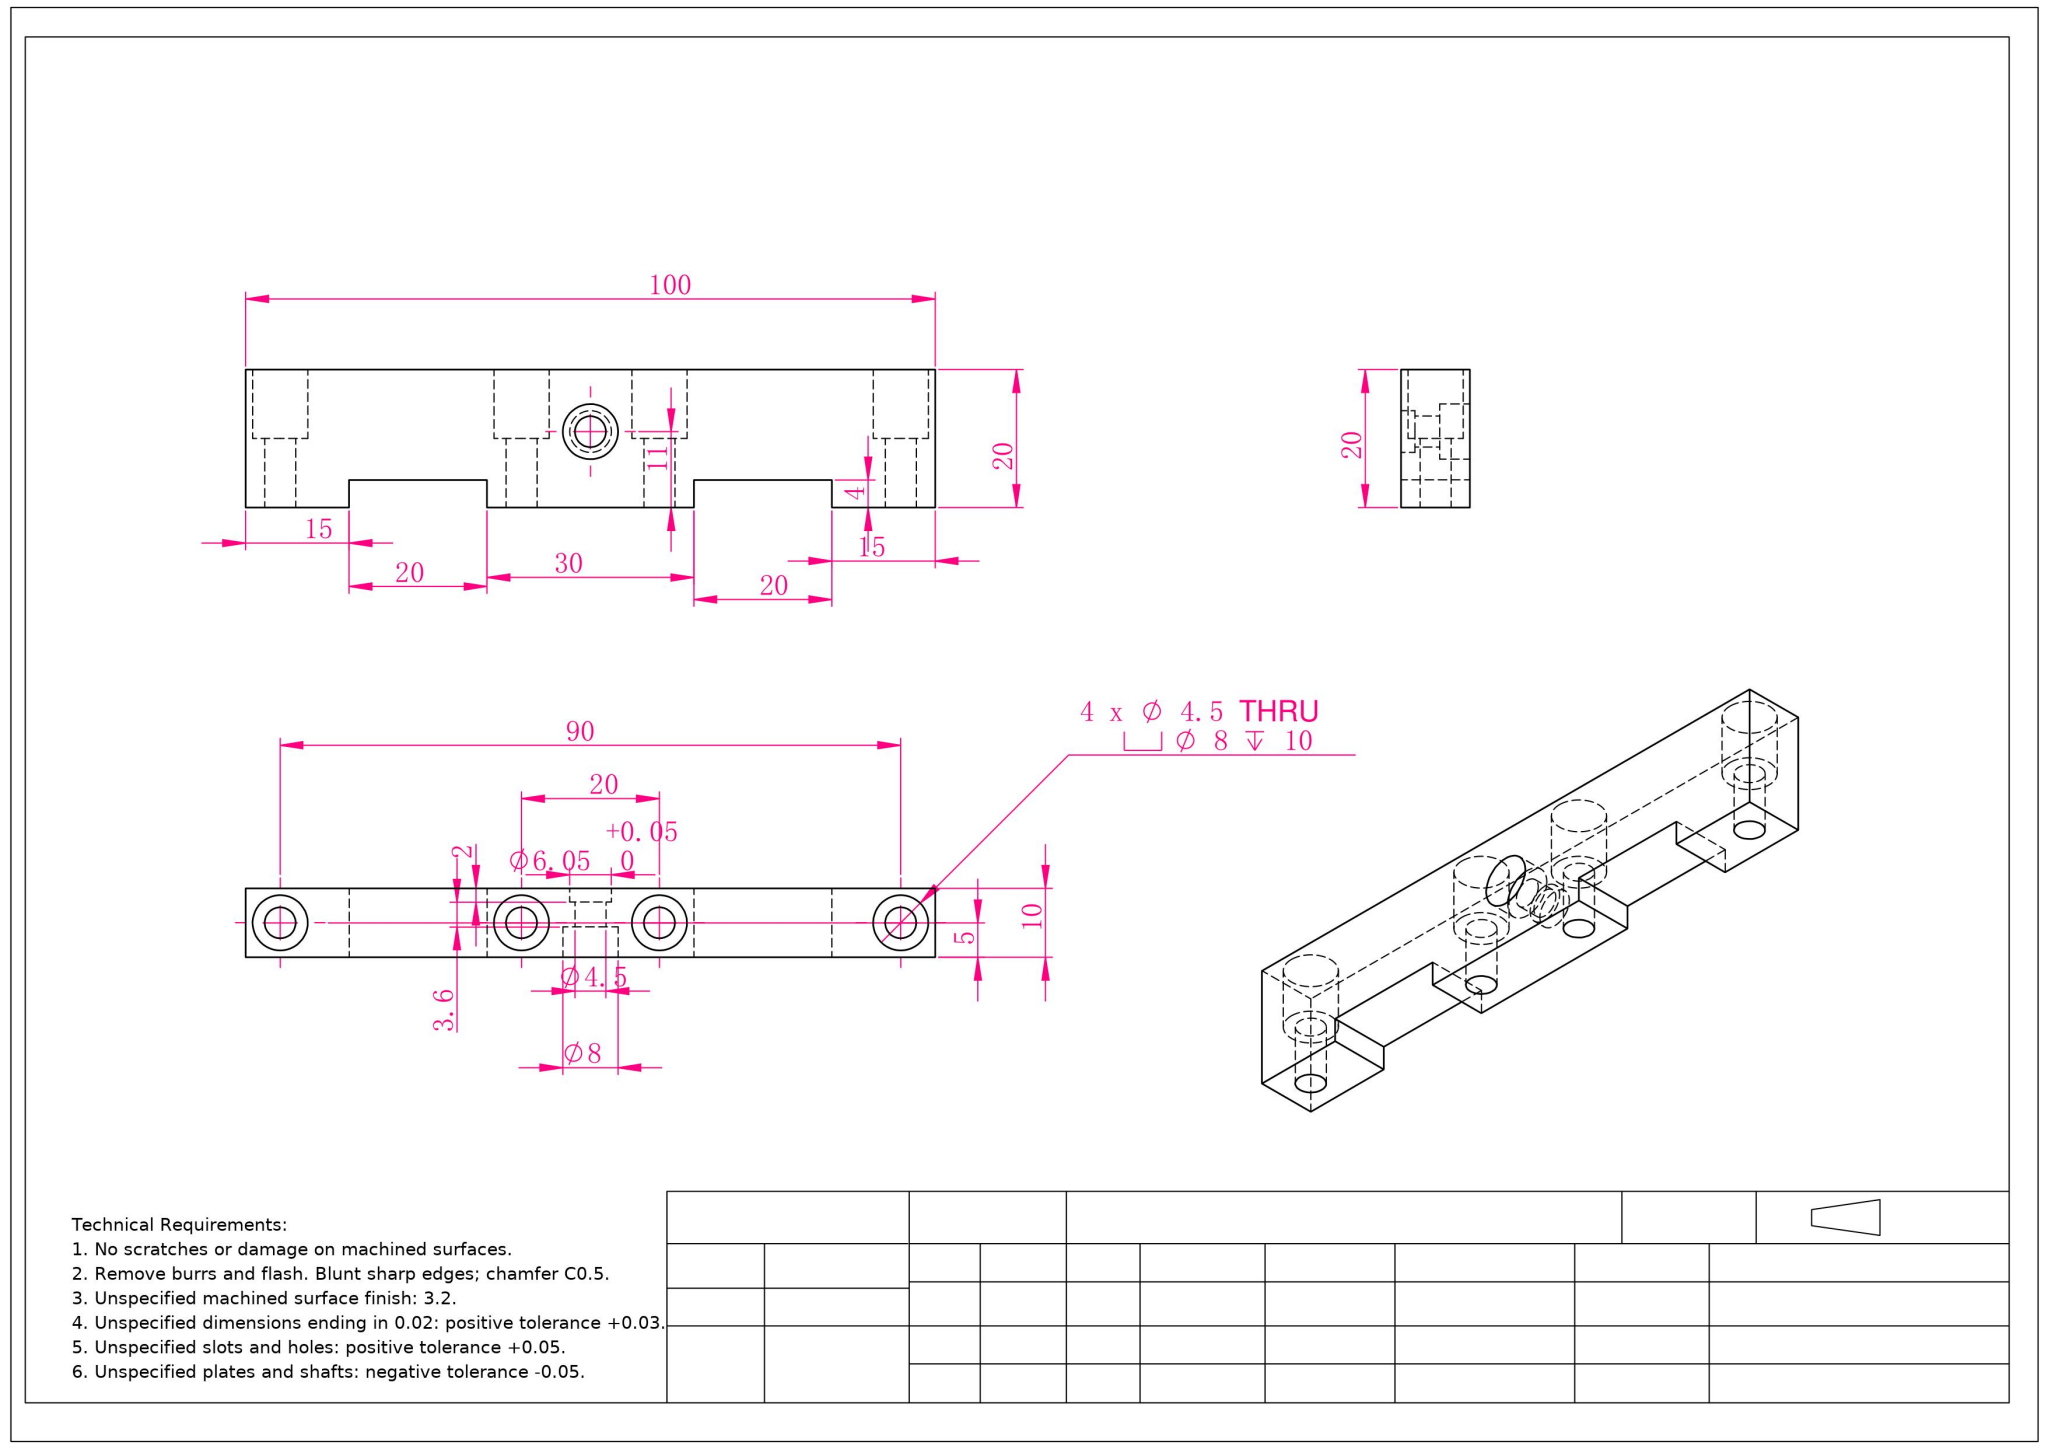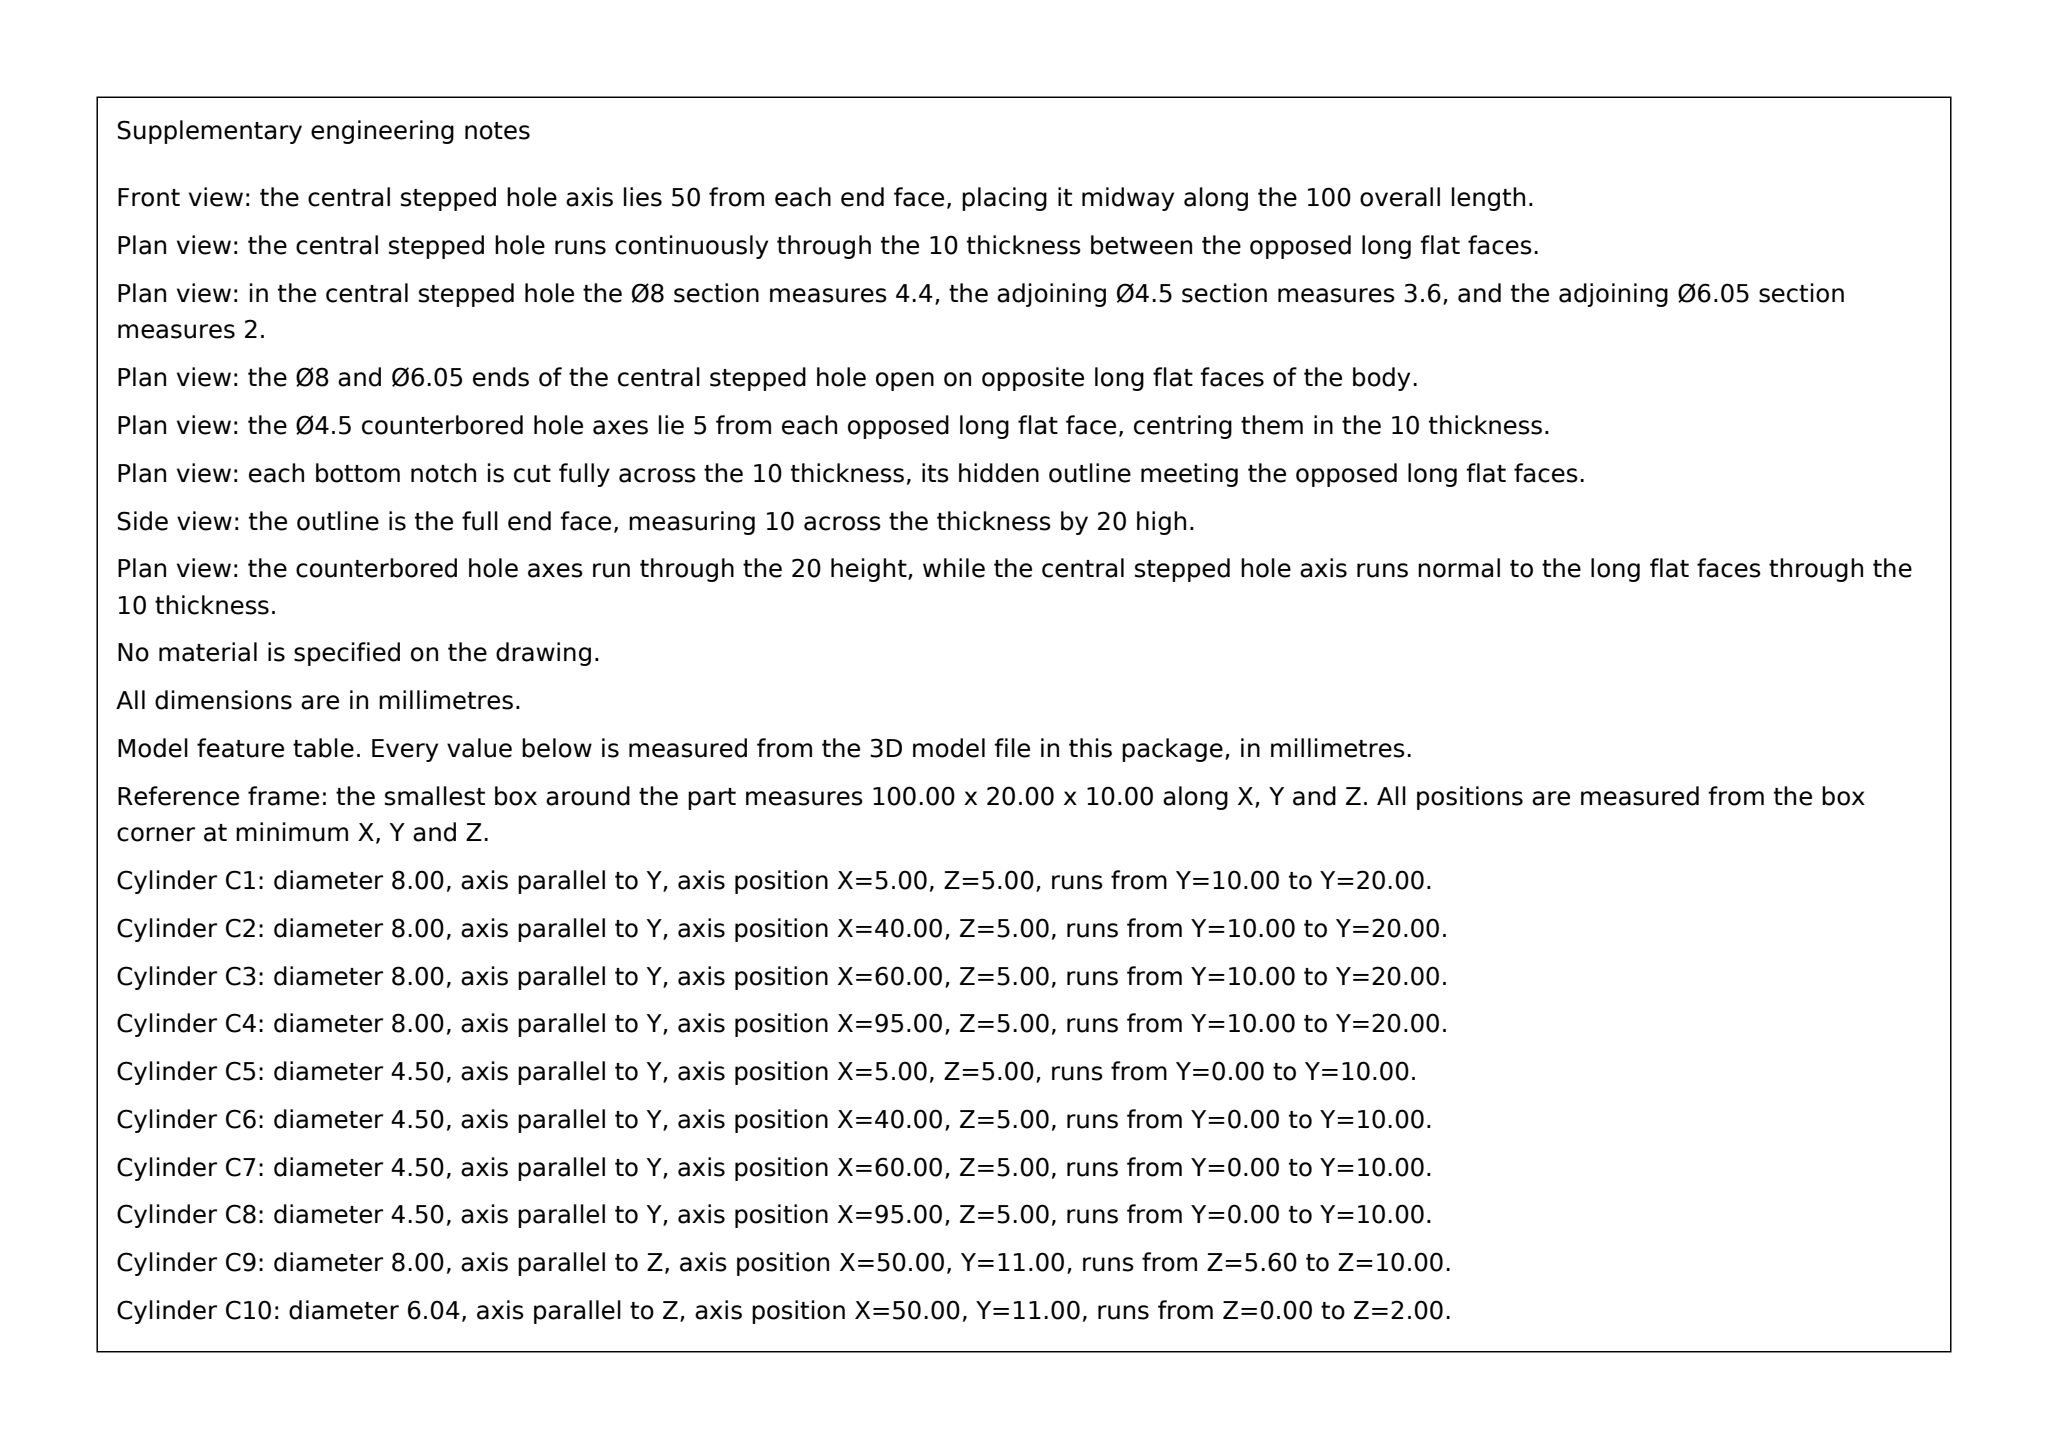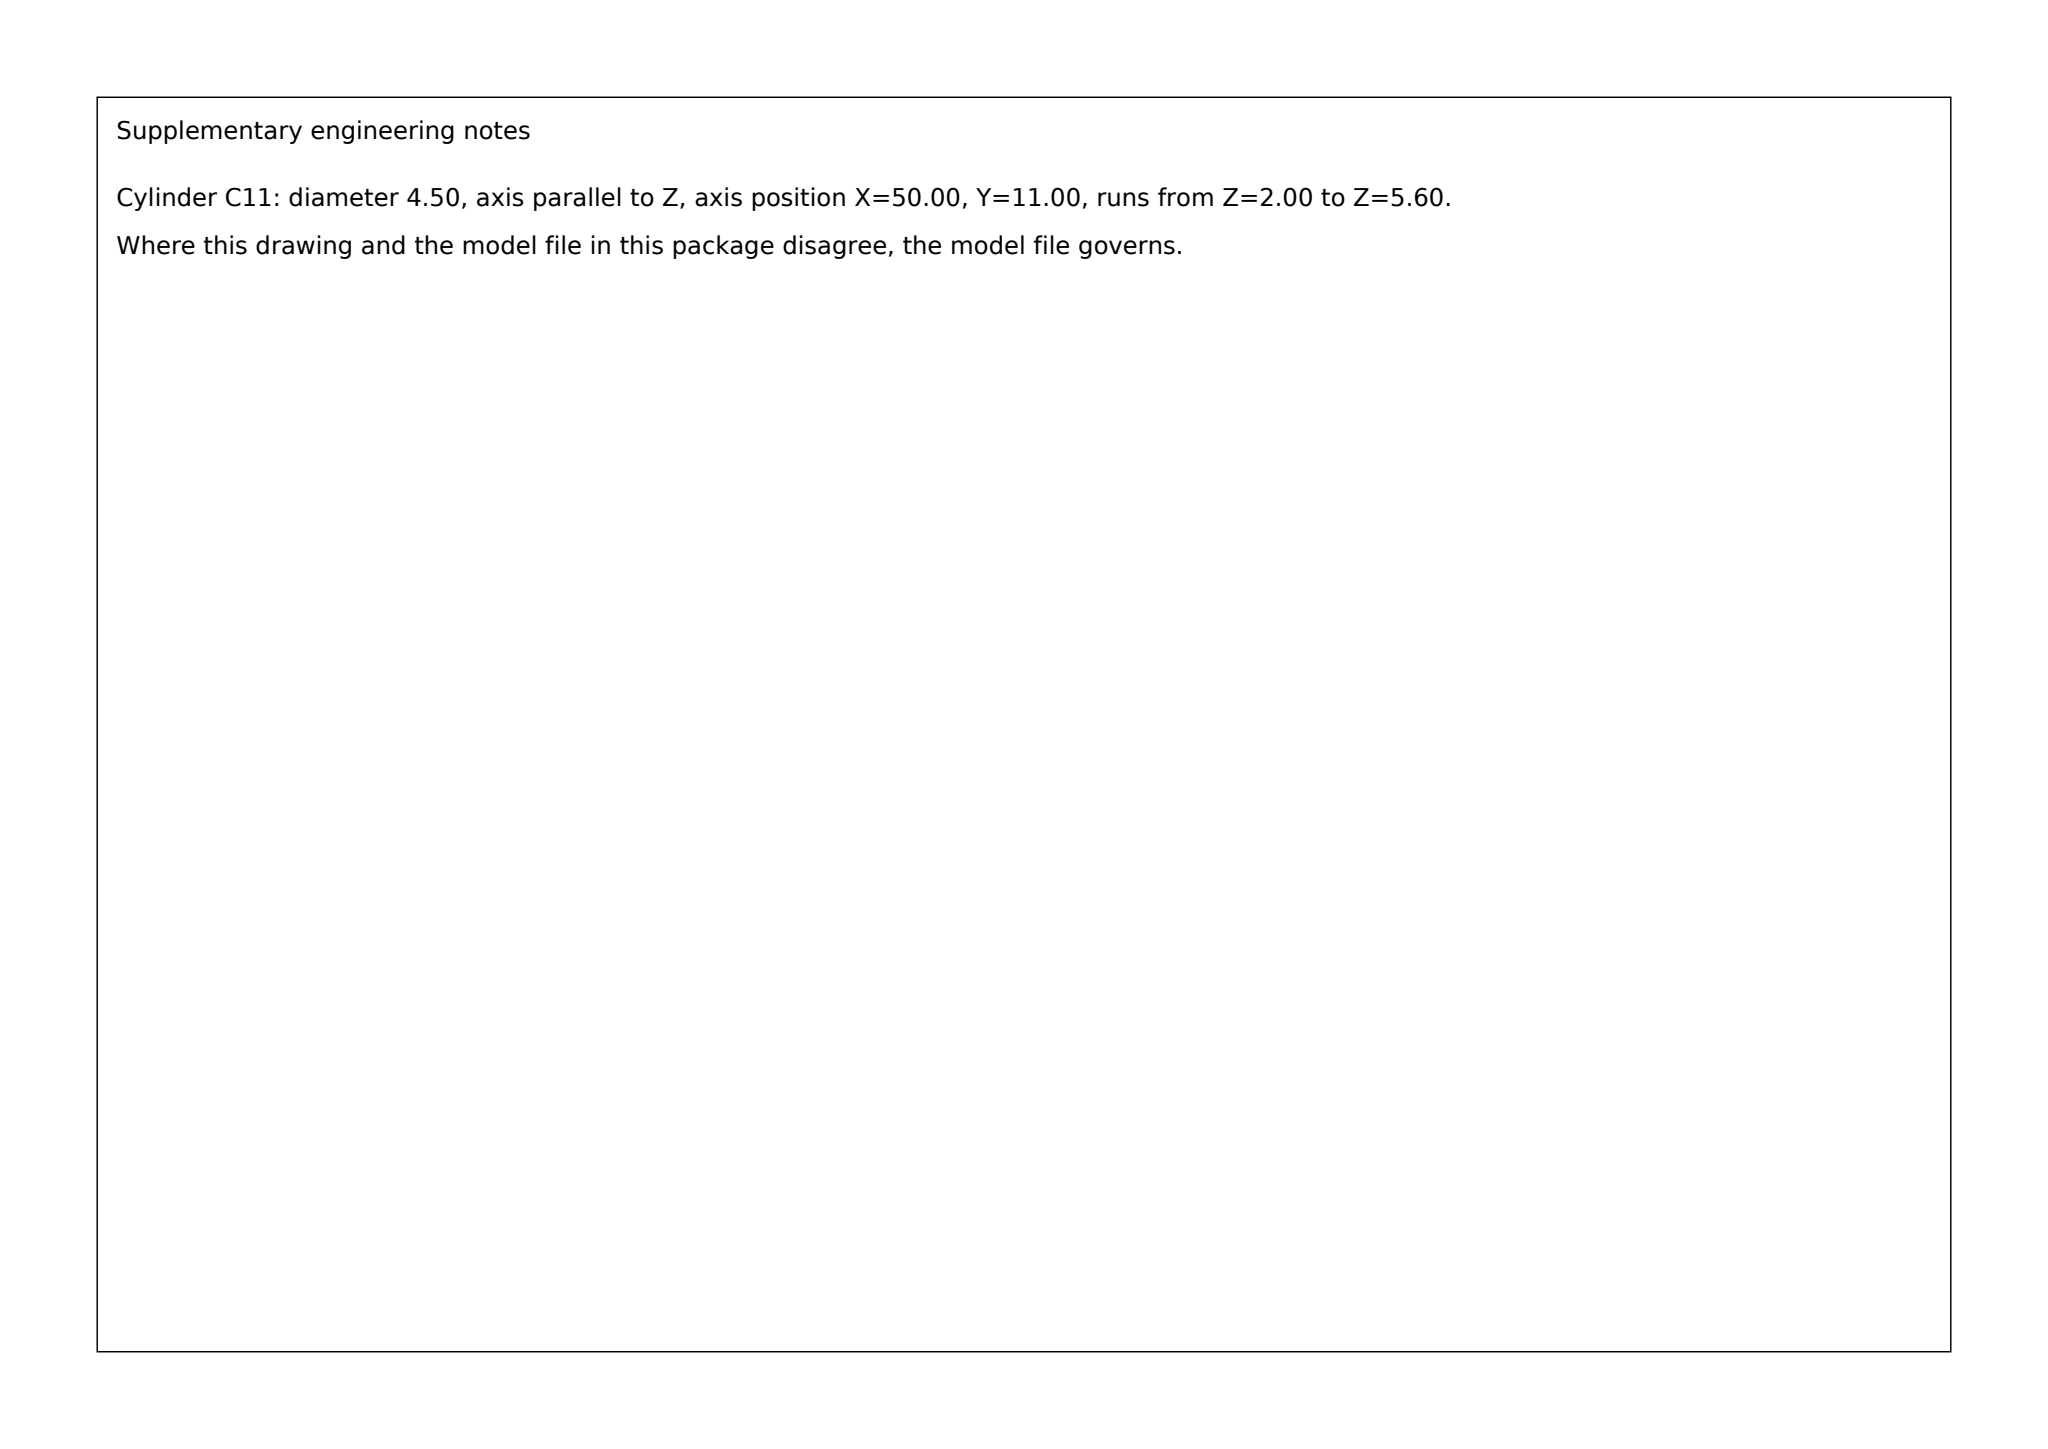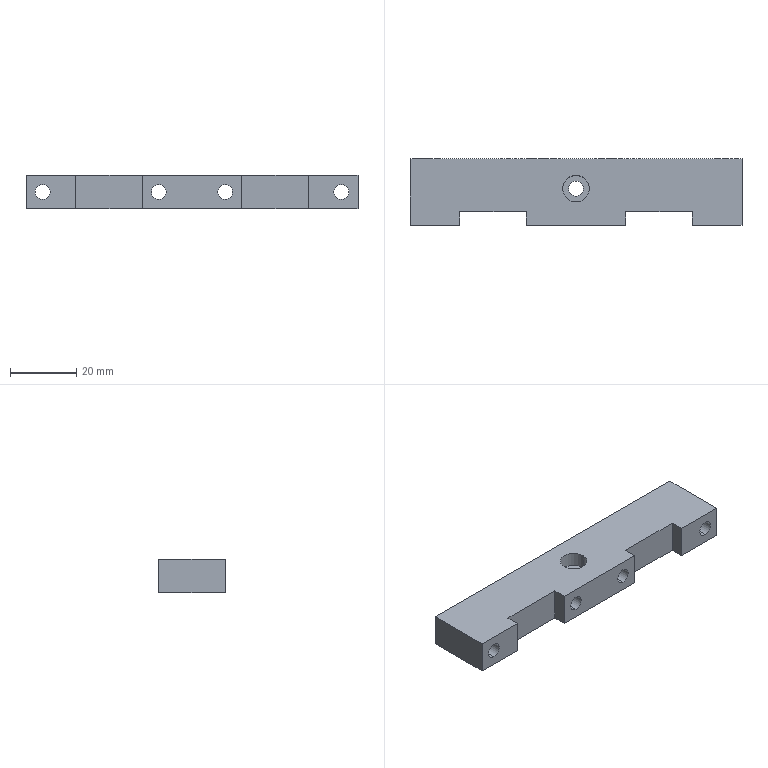Part | SolidWorks | mm | 1 solid | 42 faces | box 100 x 20 x 10 mm | volume 15417 mm3 | cylinder 22 | plane 20 | commonest cylinder face diameters 8 x10 4.5 x10 6.05 x2
build123d program:
from build123d import *

# Parameters (mm, degrees)
SKETCH1_W                                       = 100
SKETCH1_H                                       = 20
BOSS_EXTRUDE1_DEPTH                             = 5
SKETCH2_W                                       = 20
SKETCH2_H                                       = 4
CUT_EXTRUDE1_DEPTH                              = 55.772
M4_HEX_SOCKET_HEAD_CAP_SCREW_CBORE1_D           = 4.5
M4_HEX_SOCKET_HEAD_CAP_SCREW_CBORE1_CBORE_D     = 8
M4_HEX_SOCKET_HEAD_CAP_SCREW_CBORE1_CBORE_DEPTH = 4.4
SKETCH5_R                                       = 3.025
CUT_EXTRUDE2_DEPTH                              = 2
M4_HEX_SOCKET_HEAD_CAP_SCREW_CBORE2_D           = 4.5
M4_HEX_SOCKET_HEAD_CAP_SCREW_CBORE2_CBORE_D     = 8
M4_HEX_SOCKET_HEAD_CAP_SCREW_CBORE2_CBORE_DEPTH = 10


with BuildPart() as part:
    # Sketch1 → Boss-Extrude1 (new, symmetric)
    with BuildSketch(Plane.XY):
        with Locations((0, 10)):
            Rectangle(SKETCH1_W, SKETCH1_H)
    extrude(amount=BOSS_EXTRUDE1_DEPTH, both=True)

    # Sketch2 → Cut-Extrude1 (cut, through all)
    with BuildSketch(Plane.XY.offset(5)):
        with Locations((-25, 2)):
            Rectangle(SKETCH2_W, SKETCH2_H)
        with Locations((25, 2)):
            Rectangle(SKETCH2_W, SKETCH2_H)
    extrude(amount=-CUT_EXTRUDE1_DEPTH, mode=Mode.SUBTRACT)

    # M4 Hex Socket Head Cap Screw CBORE1 (through all)
    with Locations(Plane.XY.offset(5)):
        with Locations((0, 11)):
            CounterBoreHole(M4_HEX_SOCKET_HEAD_CAP_SCREW_CBORE1_D / 2, M4_HEX_SOCKET_HEAD_CAP_SCREW_CBORE1_CBORE_D / 2, M4_HEX_SOCKET_HEAD_CAP_SCREW_CBORE1_CBORE_DEPTH)

    # Sketch5 → Cut-Extrude2 (cut)
    with BuildSketch(Plane(origin=(0, 0, -5), x_dir=(-1, 0, 0), z_dir=(0, 0, -1))):
        with Locations((0, 11)):
            Circle(SKETCH5_R)
    extrude(amount=-CUT_EXTRUDE2_DEPTH, mode=Mode.SUBTRACT)

    # M4 Hex Socket Head Cap Screw CBORE2 (through all)
    with Locations(Plane(origin=(0, 20, 0), x_dir=(1, 0, 0), z_dir=(0, 1, 0))):
        with Locations((10, 0), (45, 0), (-10, 0), (-45, 0)):
            CounterBoreHole(M4_HEX_SOCKET_HEAD_CAP_SCREW_CBORE2_D / 2, M4_HEX_SOCKET_HEAD_CAP_SCREW_CBORE2_CBORE_D / 2, M4_HEX_SOCKET_HEAD_CAP_SCREW_CBORE2_CBORE_DEPTH)


solid = part.part